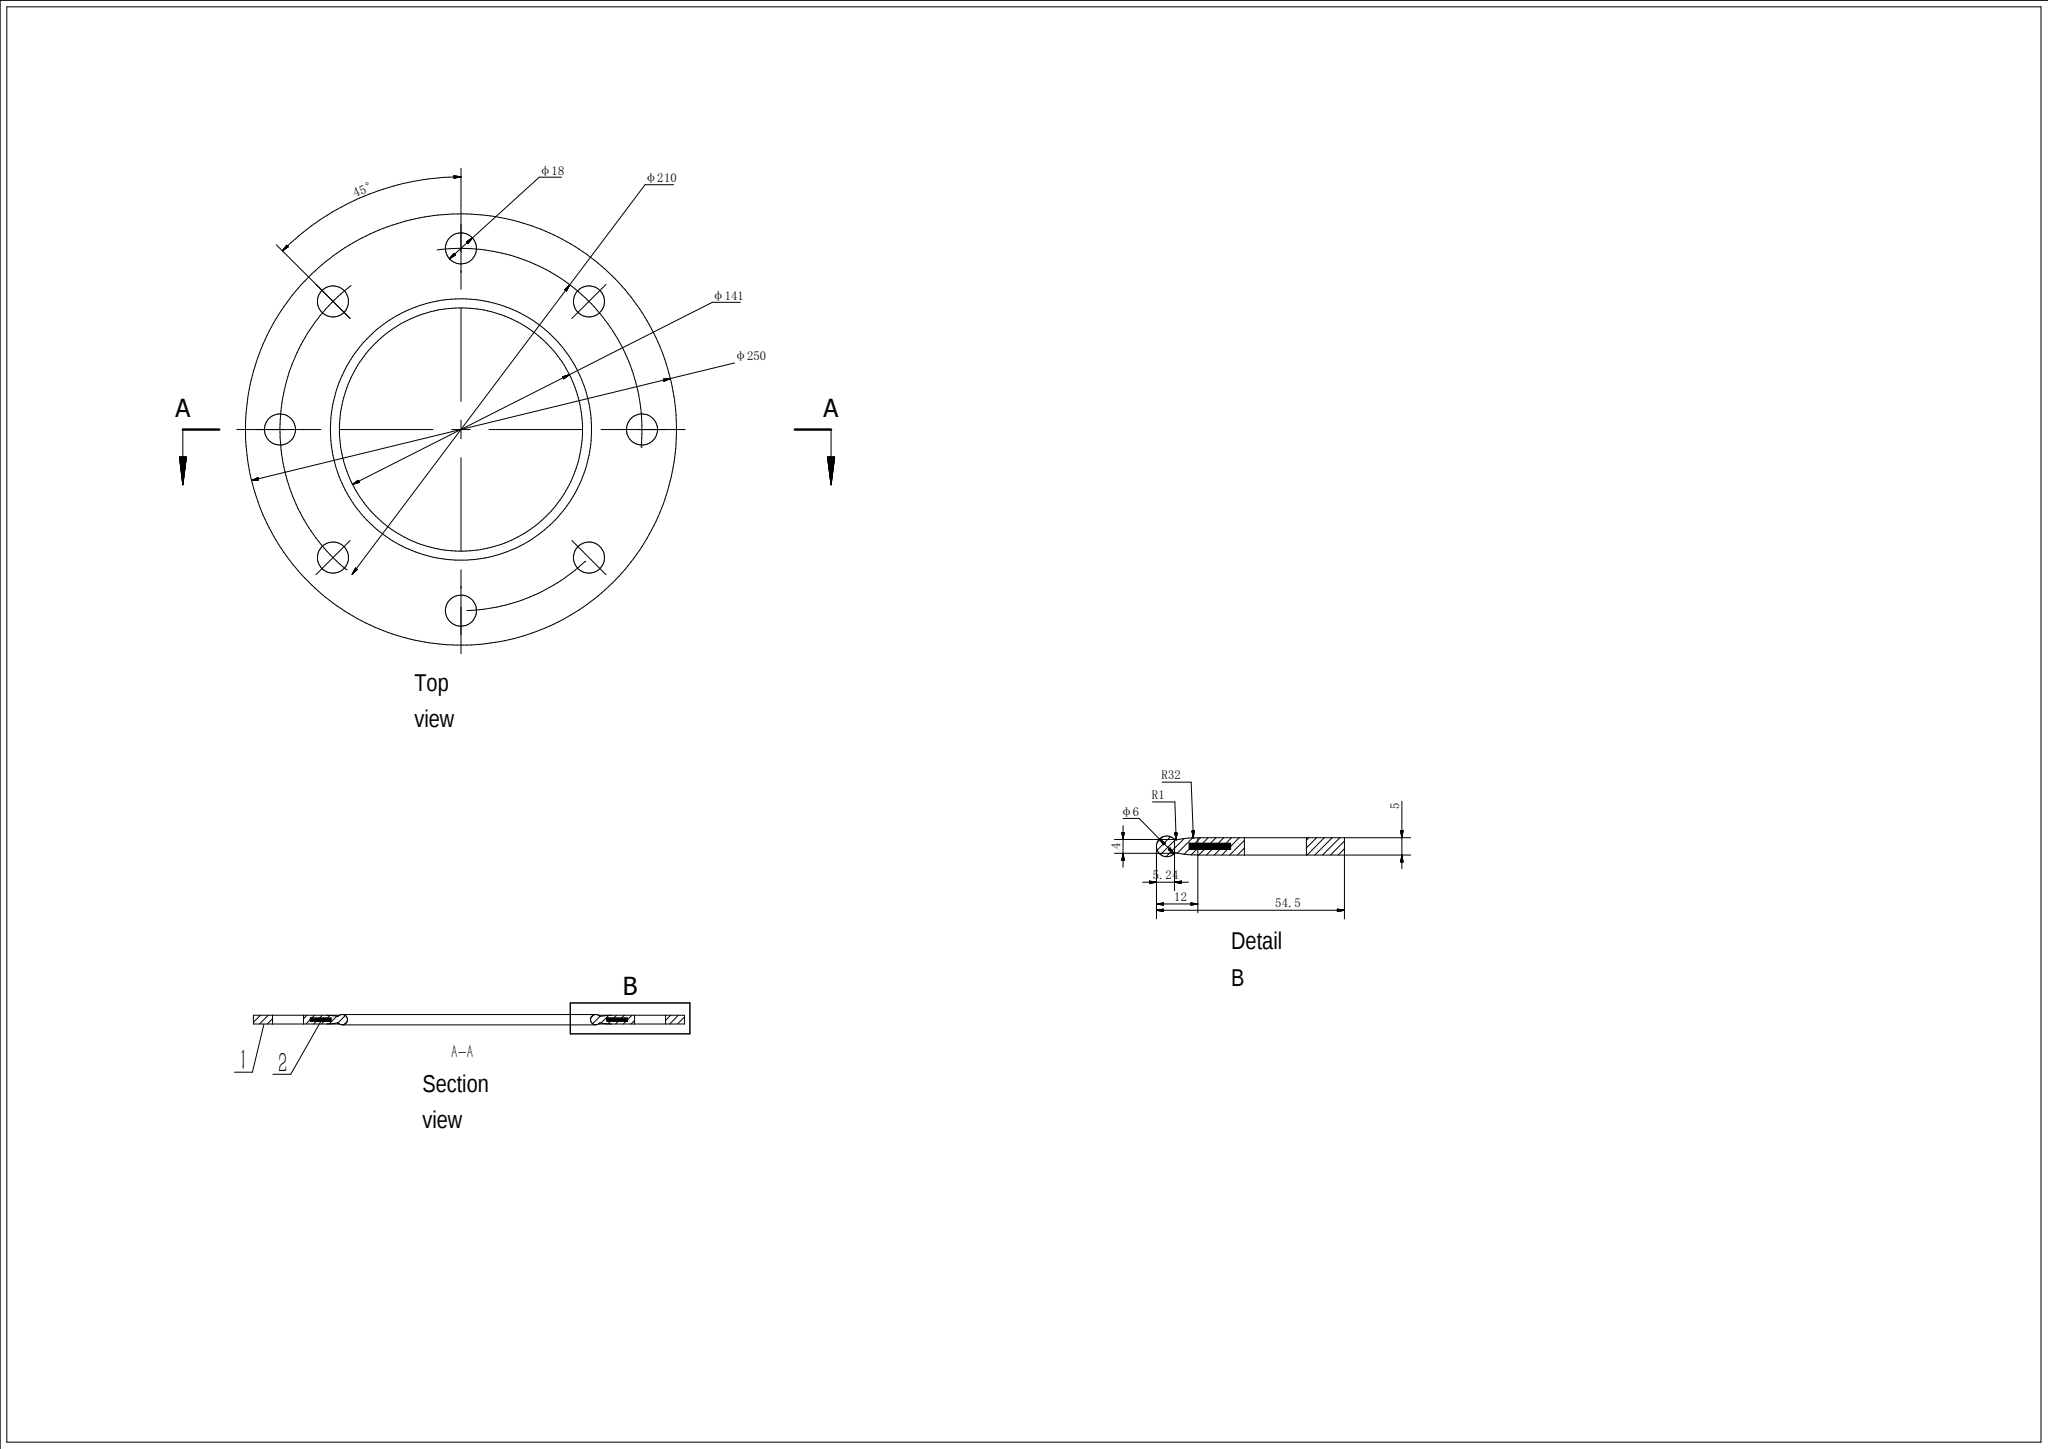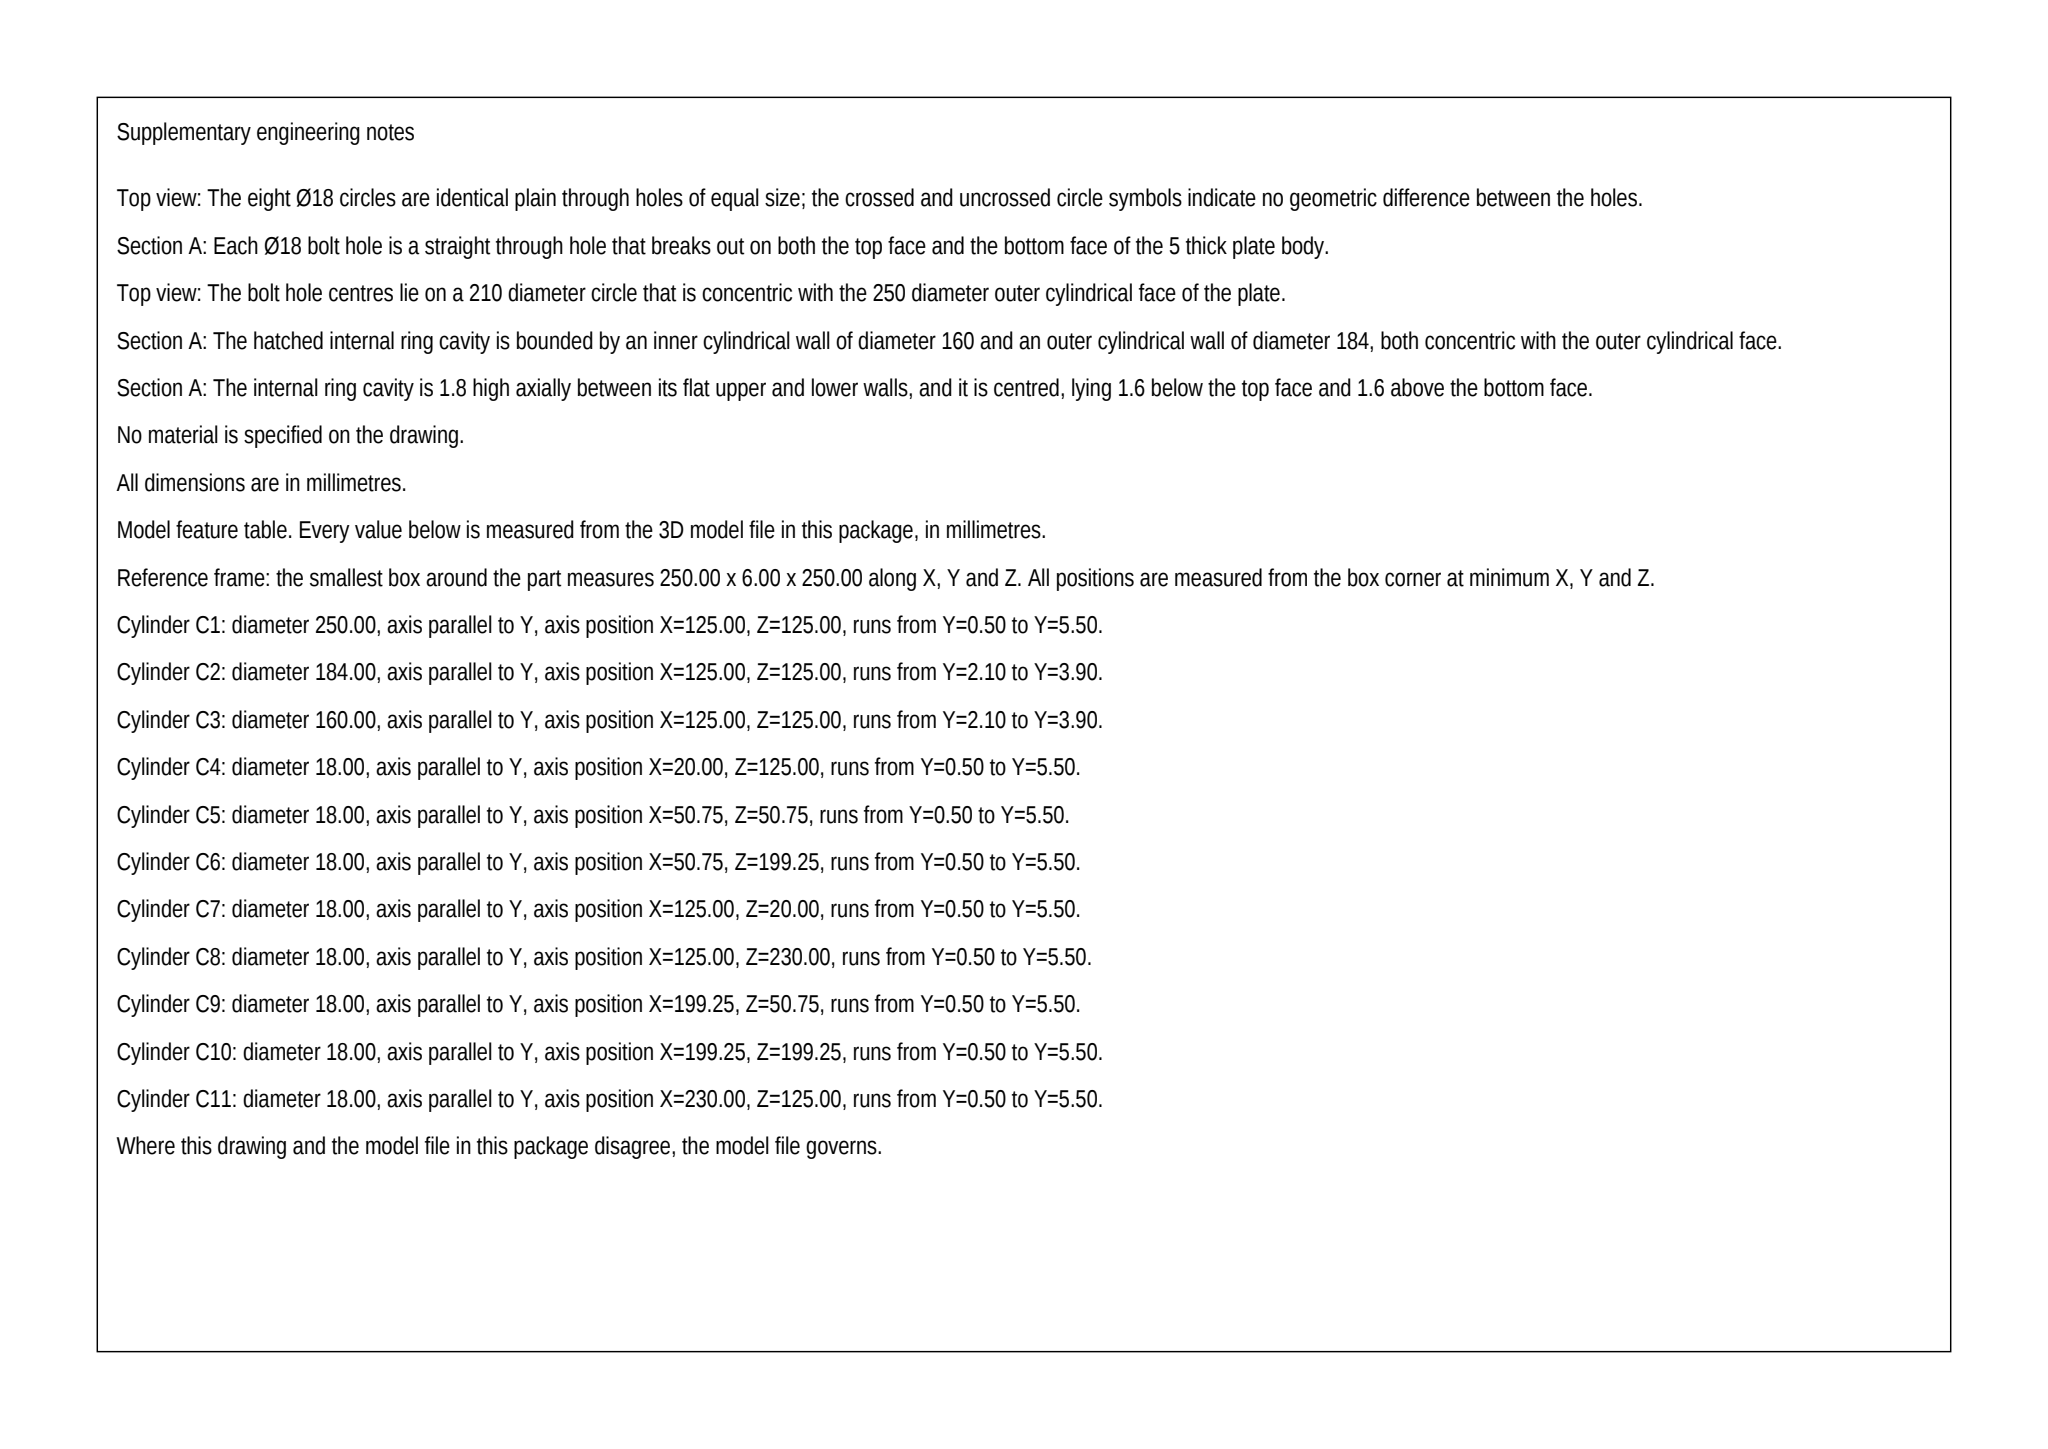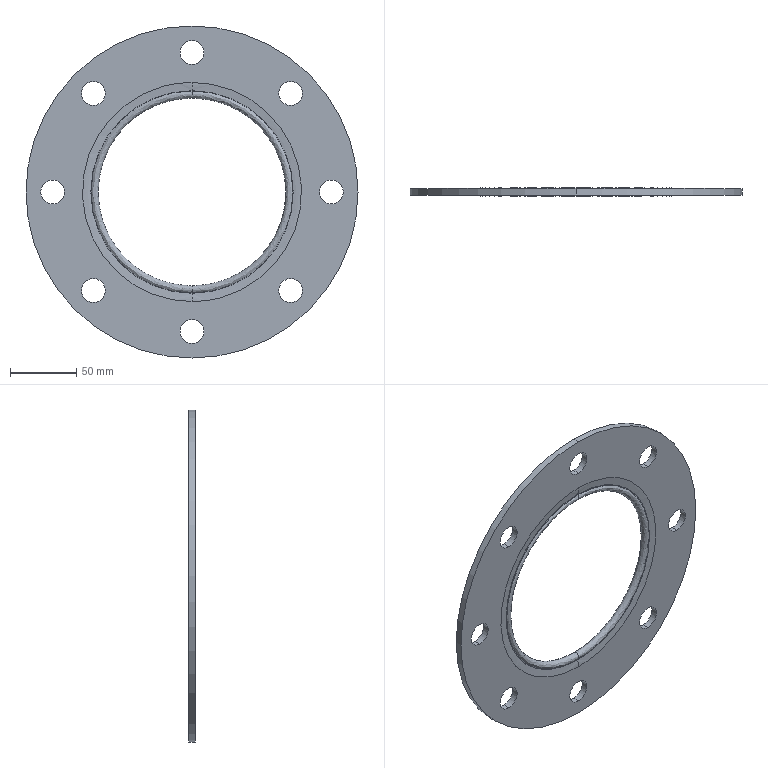Part | SolidWorks | mm | 1 solid | 36 faces | box 250 x 6 x 250 mm | volume 144077 mm3 | cylinder 22 | spline 10 | plane 4 | commonest cylinder face diameters 18 x16 250 x2 160 x2 184 x2
Drawing notes:
INNER WINDING RING Ø160, CONCENTRIC WITH Ø250 OD (COMMON CENTRE OF Ø210 BOLT CIRCLE) | from the solid: cylinder [160.0,'y',[165.0,null,125.0],1.8] shares centre with 250.0 dia cylinder at [165.0,125.0]
OUTER WINDING RING Ø184, CONCENTRIC WITH Ø250 OD (SAME CENTRE AS Ø210 BOLT CIRCLE) | from the solid: cylinder [184.0,'y',[165.0,null,125.0],1.8] shares centre with 250.0 dia cylinder at [165.0,125.0]
EACH INNER WINDING/FILLER LAYER 1.8 THK | from the solid: cylinders 160.0 and 184.0 each have length 1.8 along y
INTERNAL LAYER (Ø160 ID x Ø184 OD RING) FACES AT 1.6 AND 3.4 FROM BOTTOM FACE (DATUM A), RING 1.8 THK | from the solid: Annular ring faces are planes at y=3.5 and y=5.3 (extent x73-257, z33-217, area 6484 = Ø184/Ø160 annulus); Ø250 flange bottom face (DATUM A) is at y=1.9, so ring faces are 1.6 and 3.4 above datum, thickness 1.8
OVERALL ENVELOPE LENGTH 330.0 IN X; FLANGE RING OD Ø250 CENTRED AT X=165.0, Z=125.0 | from the solid: bbox_xyz = [330.001, 8.877, 250.001]; 250.0 dia cylinder at [165.0,null,125.0]
ALL DIMENSIONS IN MILLIMETRES (mm) UNLESS OTHERWISE STATED | from the solid: STEP model facts stated in mm
INNER SEALING/WINDING RINGS Ø160 AND Ø184, CONCENTRIC WITH Ø250 OD AND Ø210 BOLT CIRCLE (COMMON AXIS AT PART CENTRE) | from the solid: cylinders dia 160 and dia 184, axis y, pos_other_axes [165.0, 125.0] - same centre as dia 250 OD cylinder
8X Ø18 THRU 5 THK FLANGE, ON Ø210 B.C. CENTRED AT X165.0, Z125.0; HOLE AXES AT (X60.0,Z125.0), (X90.75,Z50.75), (X90.75,Z199.25), (X165.0,Z20.0), (X165.0,Z230.0), (X239.25,Z50.75), (X239.25,Z199.25), (X270.0,Z125.0) | from the solid: cylinders dia 18.0, axis y, length 5.0, eight listed positions
Ø160 AND Ø184 WINDING RING CYLINDRICAL FACES EACH 1.8 LONG IN Y, COMMON AXIS PARALLEL TO Y AT X165.0, Z125.0 | from the solid: cylinders dia 160.0 and dia 184.0, axis y, pos (165,125), length 1.8
OVERALL WIDTH 250.0 IN Z, EQUAL TO Ø250 FLANGE OD, FLANGE AXIS AT Z=125.0 (DATUM FOR Z) | from the solid: bbox_xyz Z=250.001 and Ø250 cylinder at z=125.0
OVERALL THICKNESS 8.877 IN Y FROM DATUM A (BOTTOM Ø250 FLANGE FACE), FLANGE BODY 5.0 THK, Ø160 AND Ø184 RINGS 1.8 THK EACH | from the solid: bbox_xyz Y=8.877; cylinders 250 len 5.0; cylinders 160 and 184 len 1.8
Ø160 AND Ø184 WINDING RING FACES AT 1.6 AND 3.4 FROM DATUM A (BOTTOM Ø250 FLANGE FACE), RING THK 1.8; COMMON AXIS PARALLEL TO Y AT X165.0, Z125.0 | from the solid: cylinders: boss Ø160 axis y at (165.0,125.0) from y=3.5 to 5.3 and bore Ø184 axis y at (165.0,125.0) from y=3.5 to 5.3; axis_plane y=1.9 (bottom Ø250 flange face, DATUM A) extent x[40,290] z[0,250]
Ø250 FLANGE BODY 5.0 THK: FACES AT 0.0 (DATUM A) AND 5.0, EACH SPANNING X40.0 TO X290.0 AND Z0.0 TO Z250.0 | from the solid: axis_planes y=1.9 and y=6.9, both extent x[40.0,290.0], z[0.0,250.0]; cylinder Ø250 axis y at (165.0,125.0) from y=1.9 to 6.9
ANNULAR WINDING RING: Ø160 ID x Ø184 OD x 1.8 THK, FACES AT 1.6 AND 3.4 FROM DATUM A (BOTTOM Ø250 FLANGE FACE), AXIS PARALLEL TO Y AT X165.0, Z125.0 | from the solid: cylinders boss Ø160 and bore Ø184 on y axis at (165,125) from y3.5 to y5.3; axis_planes y=3.5 and y=5.3, extent x[73,257] z[33,217], area 6484 (annulus Ø160/Ø184)
Ø250 x 5.0 THK FLANGE BODY LIES BETWEEN Y=1.9 AND Y=6.9 FROM MIN CORNER OF THE 8.877 OVERALL ENVELOPE; NO OTHER MATERIAL IS MODELLED BELOW Y=1.9 OR ABOVE Y=6.9 | from the solid: cylinder boss Ø250 on y axis at (165,125) from 1.9 to 6.9; bbox_xyz y = 8.877
Ø250 FLANGE BODY FACES SPAN X40.0 TO X290.0 AND Z0.0 TO Z250.0; NO MODELLED MATERIAL IN X0 TO X40.0 OR X290.0 TO X330.0 OF THE 330.0 ENVELOPE | from the solid: axis_planes y=1.9 and y=6.9, extent x[40.0,290.0] z[0.0,250.0], area 25690; bbox_xyz x = 330.001